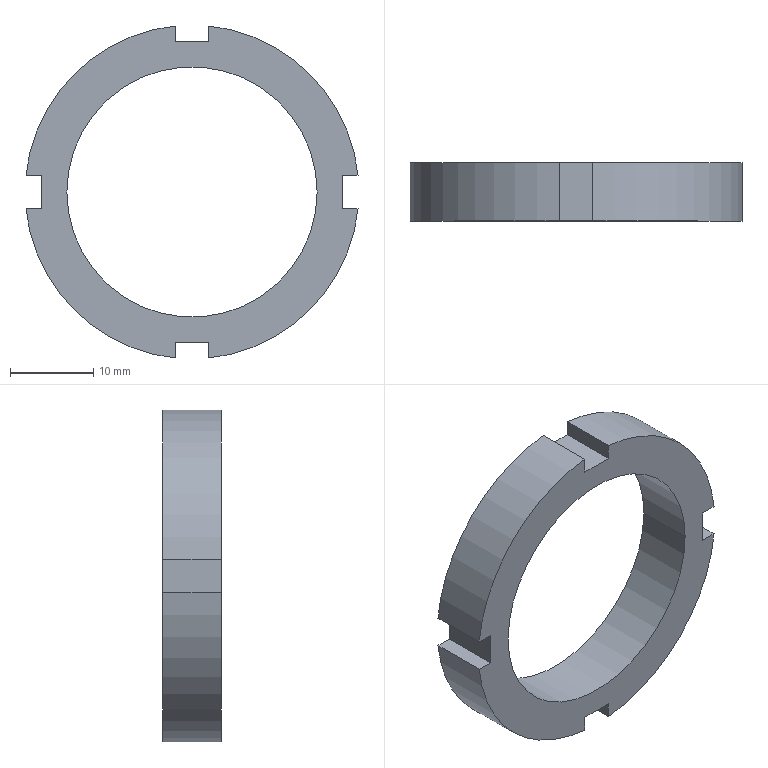Component | SolidWorks | -M30X1.5Nut-1 | 1 solid | 20 faces | box 39.8 x 7 x 39.8 mm | volume 3628 mm3 | plane 14 | cylinder 6 | commonest cylinder face diameters 40 x4 30 x2
build123d program:
from build123d import *

# Parameters (mm, degrees)
BOSS_EXTRUDE1_DEPTH        = 3.5
M30X2_0_TAPPED_HOLE1_D     = 30
M30X2_0_TAPPED_HOLE1_DEPTH = 70
M30X2_0_TAPPED_HOLE1_TIP   = 9.013


with BuildPart() as part:
    # Sketch1 → Boss-Extrude1 (new, symmetric)
    with BuildSketch(Plane.XY):
        with BuildLine():
            Line((2, 18), (2, 19.9))
            ThreePointArc((2, 19.9), (14.142, 14.142), (19.9, 2))
            Line((19.9, 2), (18, 2))
            Line((18, 2), (18, -2))
            Line((18, -2), (19.9, -2))
            ThreePointArc((19.9, -2), (14.142, -14.142), (2, -19.9))
            Line((2, -19.9), (2, -18))
            Line((2, -18), (-2, -18))
            Line((-2, -18), (-2, -19.9))
            ThreePointArc((-2, -19.9), (-14.142, -14.142), (-19.9, -2))
            Line((-19.9, -2), (-18, -2))
            Line((-18, -2), (-18, 2))
            Line((-18, 2), (-19.9, 2))
            ThreePointArc((-19.9, 2), (-14.142, 14.142), (-2, 19.9))
            Line((-2, 19.9), (-2, 18))
            Line((-2, 18), (2, 18))
        make_face()
    extrude(amount=BOSS_EXTRUDE1_DEPTH, both=True)

    # M30x2.0 Tapped Hole1
    with Locations(Plane.XY.offset(3.5)):
        with Locations((0, 0)):
            Hole(M30X2_0_TAPPED_HOLE1_D / 2, depth=M30X2_0_TAPPED_HOLE1_DEPTH)
            with Locations((0, 0, -(M30X2_0_TAPPED_HOLE1_DEPTH + M30X2_0_TAPPED_HOLE1_TIP / 2))):  # 118° drill point
                Cone(0, M30X2_0_TAPPED_HOLE1_D / 2, M30X2_0_TAPPED_HOLE1_TIP, mode=Mode.SUBTRACT)


solid = part.part

# Placed as in the assembly
solid = solid.moved(Location((205, 1325, -173), (90, 0, 0)))
STEP:
#1=COLOUR_RGB('',0.7922,0.8196,0.9333);
#2=FILL_AREA_STYLE_COLOUR('',#1);
#3=FILL_AREA_STYLE('',(#2));
#4=SURFACE_STYLE_FILL_AREA(#3);
#5=SURFACE_SIDE_STYLE('',(#4));
#6=SURFACE_STYLE_USAGE(.BOTH.,#5);
#7=PRESENTATION_STYLE_ASSIGNMENT((#6));
#8=CARTESIAN_POINT('',(7.48,52.303,-6.811));
#9=VERTEX_POINT('',#8);
#10=CARTESIAN_POINT('',(8.661,52.303,-6.811));
#11=VERTEX_POINT('',#10);
#12=CARTESIAN_POINT('',(8.071,52.303,-6.811));
#13=DIRECTION('',(0.,-1.,0.));
#14=DIRECTION('',(1.,0.,0.));
#15=AXIS2_PLACEMENT_3D('',#12,#13,#14);
#16=CIRCLE('',#15,0.5906);
#17=EDGE_CURVE('',#9,#11,#16,.T.);
#18=ORIENTED_EDGE('',*,*,#17,.F.);
#19=CARTESIAN_POINT('',(7.48,52.028,-6.811));
#20=VERTEX_POINT('',#19);
#21=CARTESIAN_POINT('',(7.48,52.028,-6.811));
#22=DIRECTION('',(0.,-1.,0.));
#23=VECTOR('',#22,39.37);
#24=LINE('',#21,#23);
#25=EDGE_CURVE('',#9,#20,#24,.T.);
#26=ORIENTED_EDGE('',*,*,#25,.T.);
#27=CARTESIAN_POINT('',(8.661,52.028,-6.811));
#28=VERTEX_POINT('',#27);
#29=CARTESIAN_POINT('',(8.071,52.028,-6.811));
#30=DIRECTION('',(0.,-1.,0.));
#31=DIRECTION('',(1.,0.,0.));
#32=AXIS2_PLACEMENT_3D('',#29,#30,#31);
#33=CIRCLE('',#32,0.5906);
#34=EDGE_CURVE('',#20,#28,#33,.T.);
#35=ORIENTED_EDGE('',*,*,#34,.T.);
#36=CARTESIAN_POINT('',(8.661,52.028,-6.811));
#37=DIRECTION('',(0.,-1.,0.));
#38=VECTOR('',#37,39.37);
#39=LINE('',#36,#38);
#40=EDGE_CURVE('',#11,#28,#39,.T.);
#41=ORIENTED_EDGE('',*,*,#40,.F.);
#42=EDGE_LOOP('',(#18,#26,#35,#41));
#43=FACE_OUTER_BOUND('',#42,.T.);
#44=CARTESIAN_POINT('',(8.071,52.028,-6.811));
#45=DIRECTION('',(0.,-1.,0.));
#46=DIRECTION('',(1.,0.,0.));
#47=AXIS2_PLACEMENT_3D('',#44,#45,#46);
#48=CYLINDRICAL_SURFACE('',#47,0.5906);
#49=ADVANCED_FACE('',(#43),#48,.F.);
#50=CARTESIAN_POINT('',(8.854,52.303,-6.732));
#51=VERTEX_POINT('',#50);
#52=CARTESIAN_POINT('',(8.15,52.303,-6.028));
#53=VERTEX_POINT('',#52);
#54=CARTESIAN_POINT('',(8.071,52.303,-6.811));
#55=DIRECTION('',(0.,-1.,0.));
#56=DIRECTION('',(1.,0.,0.));
#57=AXIS2_PLACEMENT_3D('',#54,#55,#56);
#58=CIRCLE('',#57,0.7874);
#59=EDGE_CURVE('',#51,#53,#58,.T.);
#60=ORIENTED_EDGE('',*,*,#59,.T.);
#61=CARTESIAN_POINT('',(8.15,52.028,-6.028));
#62=VERTEX_POINT('',#61);
#63=CARTESIAN_POINT('',(8.15,52.028,-6.028));
#64=DIRECTION('',(-0.,1.,-0.));
#65=VECTOR('',#64,39.37);
#66=LINE('',#63,#65);
#67=EDGE_CURVE('',#62,#53,#66,.T.);
#68=ORIENTED_EDGE('',*,*,#67,.F.);
#69=CARTESIAN_POINT('',(8.854,52.028,-6.732));
#70=VERTEX_POINT('',#69);
#71=CARTESIAN_POINT('',(8.071,52.028,-6.811));
#72=DIRECTION('',(0.,-1.,0.));
#73=DIRECTION('',(1.,0.,0.));
#74=AXIS2_PLACEMENT_3D('',#71,#72,#73);
#75=CIRCLE('',#74,0.7874);
#76=EDGE_CURVE('',#70,#62,#75,.T.);
#77=ORIENTED_EDGE('',*,*,#76,.F.);
#78=CARTESIAN_POINT('',(8.854,52.028,-6.732));
#79=DIRECTION('',(-0.,1.,-0.));
#80=VECTOR('',#79,39.37);
#81=LINE('',#78,#80);
#82=EDGE_CURVE('',#70,#51,#81,.T.);
#83=ORIENTED_EDGE('',*,*,#82,.T.);
#84=EDGE_LOOP('',(#60,#68,#77,#83));
#85=FACE_OUTER_BOUND('',#84,.T.);
#86=CARTESIAN_POINT('',(8.071,52.028,-6.811));
#87=DIRECTION('',(-0.,1.,-0.));
#88=DIRECTION('',(-1.,0.,0.));
#89=AXIS2_PLACEMENT_3D('',#86,#87,#88);
#90=CYLINDRICAL_SURFACE('',#89,0.7874);
#91=ADVANCED_FACE('',(#85),#90,.T.);
#92=CARTESIAN_POINT('',(8.15,52.303,-6.102));
#93=VERTEX_POINT('',#92);
#94=CARTESIAN_POINT('',(8.15,52.303,-6.102));
#95=DIRECTION('',(-0.,-0.,-1.));
#96=VECTOR('',#95,39.37);
#97=LINE('',#94,#96);
#98=EDGE_CURVE('',#53,#93,#97,.T.);
#99=ORIENTED_EDGE('',*,*,#98,.T.);
#100=CARTESIAN_POINT('',(8.15,52.028,-6.102));
#101=VERTEX_POINT('',#100);
#102=CARTESIAN_POINT('',(8.15,52.028,-6.102));
#103=DIRECTION('',(-0.,1.,-0.));
#104=VECTOR('',#103,39.37);
#105=LINE('',#102,#104);
#106=EDGE_CURVE('',#101,#93,#105,.T.);
#107=ORIENTED_EDGE('',*,*,#106,.F.);
#108=CARTESIAN_POINT('',(8.15,52.028,-6.102));
#109=DIRECTION('',(-0.,-0.,-1.));
#110=VECTOR('',#109,39.37);
#111=LINE('',#108,#110);
#112=EDGE_CURVE('',#62,#101,#111,.T.);
#113=ORIENTED_EDGE('',*,*,#112,.F.);
#114=ORIENTED_EDGE('',*,*,#67,.T.);
#115=EDGE_LOOP('',(#99,#107,#113,#114));
#116=FACE_OUTER_BOUND('',#115,.T.);
#117=CARTESIAN_POINT('',(8.15,52.028,-6.102));
#118=DIRECTION('',(1.,0.,-0.));
#119=DIRECTION('',(-0.,1.,-0.));
#120=AXIS2_PLACEMENT_3D('',#117,#118,#119);
#121=PLANE('',#120);
#122=ADVANCED_FACE('',(#116),#121,.F.);
#123=CARTESIAN_POINT('',(7.992,52.303,-6.102));
#124=VERTEX_POINT('',#123);
#125=CARTESIAN_POINT('',(7.992,52.303,-6.102));
#126=DIRECTION('',(-1.,-0.,0.));
#127=VECTOR('',#126,39.37);
#128=LINE('',#125,#127);
#129=EDGE_CURVE('',#93,#124,#128,.T.);
#130=ORIENTED_EDGE('',*,*,#129,.T.);
#131=CARTESIAN_POINT('',(7.992,52.028,-6.102));
#132=VERTEX_POINT('',#131);
#133=CARTESIAN_POINT('',(7.992,52.028,-6.102));
#134=DIRECTION('',(-0.,1.,-0.));
#135=VECTOR('',#134,39.37);
#136=LINE('',#133,#135);
#137=EDGE_CURVE('',#132,#124,#136,.T.);
#138=ORIENTED_EDGE('',*,*,#137,.F.);
#139=CARTESIAN_POINT('',(7.992,52.028,-6.102));
#140=DIRECTION('',(-1.,-0.,0.));
#141=VECTOR('',#140,39.37);
#142=LINE('',#139,#141);
#143=EDGE_CURVE('',#101,#132,#142,.T.);
#144=ORIENTED_EDGE('',*,*,#143,.F.);
#145=ORIENTED_EDGE('',*,*,#106,.T.);
#146=EDGE_LOOP('',(#130,#138,#144,#145));
#147=FACE_OUTER_BOUND('',#146,.T.);
#148=CARTESIAN_POINT('',(7.992,52.028,-6.102));
#149=DIRECTION('',(-0.,-0.,-1.));
#150=DIRECTION('',(-0.,1.,-0.));
#151=AXIS2_PLACEMENT_3D('',#148,#149,#150);
#152=PLANE('',#151);
#153=ADVANCED_FACE('',(#147),#152,.F.);
#154=CARTESIAN_POINT('',(7.992,52.303,-6.028));
#155=VERTEX_POINT('',#154);
#156=CARTESIAN_POINT('',(7.992,52.303,-6.102));
#157=DIRECTION('',(0.,0.,1.));
#158=VECTOR('',#157,39.37);
#159=LINE('',#156,#158);
#160=EDGE_CURVE('',#124,#155,#159,.T.);
#161=ORIENTED_EDGE('',*,*,#160,.T.);
#162=CARTESIAN_POINT('',(7.992,52.028,-6.028));
#163=VERTEX_POINT('',#162);
#164=CARTESIAN_POINT('',(7.992,52.028,-6.028));
#165=DIRECTION('',(-0.,1.,-0.));
#166=VECTOR('',#165,39.37);
#167=LINE('',#164,#166);
#168=EDGE_CURVE('',#163,#155,#167,.T.);
#169=ORIENTED_EDGE('',*,*,#168,.F.);
#170=CARTESIAN_POINT('',(7.992,52.028,-6.102));
#171=DIRECTION('',(0.,0.,1.));
#172=VECTOR('',#171,39.37);
#173=LINE('',#170,#172);
#174=EDGE_CURVE('',#132,#163,#173,.T.);
#175=ORIENTED_EDGE('',*,*,#174,.F.);
#176=ORIENTED_EDGE('',*,*,#137,.T.);
#177=EDGE_LOOP('',(#161,#169,#175,#176));
#178=FACE_OUTER_BOUND('',#177,.T.);
#179=CARTESIAN_POINT('',(7.992,52.028,-6.102));
#180=DIRECTION('',(-1.,-0.,0.));
#181=DIRECTION('',(0.,-1.,0.));
#182=AXIS2_PLACEMENT_3D('',#179,#180,#181);
#183=PLANE('',#182);
#184=ADVANCED_FACE('',(#178),#183,.F.);
#185=CARTESIAN_POINT('',(7.287,52.303,-6.732));
#186=VERTEX_POINT('',#185);
#187=CARTESIAN_POINT('',(8.071,52.303,-6.811));
#188=DIRECTION('',(0.,-1.,0.));
#189=DIRECTION('',(1.,0.,0.));
#190=AXIS2_PLACEMENT_3D('',#187,#188,#189);
#191=CIRCLE('',#190,0.7874);
#192=EDGE_CURVE('',#155,#186,#191,.T.);
#193=ORIENTED_EDGE('',*,*,#192,.T.);
#194=CARTESIAN_POINT('',(7.287,52.028,-6.732));
#195=VERTEX_POINT('',#194);
#196=CARTESIAN_POINT('',(7.287,52.028,-6.732));
#197=DIRECTION('',(-0.,1.,-0.));
#198=VECTOR('',#197,39.37);
#199=LINE('',#196,#198);
#200=EDGE_CURVE('',#195,#186,#199,.T.);
#201=ORIENTED_EDGE('',*,*,#200,.F.);
#202=CARTESIAN_POINT('',(8.071,52.028,-6.811));
#203=DIRECTION('',(0.,-1.,0.));
#204=DIRECTION('',(1.,0.,0.));
#205=AXIS2_PLACEMENT_3D('',#202,#203,#204);
#206=CIRCLE('',#205,0.7874);
#207=EDGE_CURVE('',#163,#195,#206,.T.);
#208=ORIENTED_EDGE('',*,*,#207,.F.);
#209=ORIENTED_EDGE('',*,*,#168,.T.);
#210=EDGE_LOOP('',(#193,#201,#208,#209));
#211=FACE_OUTER_BOUND('',#210,.T.);
#212=CARTESIAN_POINT('',(8.071,52.028,-6.811));
#213=DIRECTION('',(-0.,1.,-0.));
#214=DIRECTION('',(-1.,0.,0.));
#215=AXIS2_PLACEMENT_3D('',#212,#213,#214);
#216=CYLINDRICAL_SURFACE('',#215,0.7874);
#217=ADVANCED_FACE('',(#211),#216,.T.);
#218=CARTESIAN_POINT('',(7.362,52.303,-6.732));
#219=VERTEX_POINT('',#218);
#220=CARTESIAN_POINT('',(7.362,52.303,-6.732));
#221=DIRECTION('',(1.,0.,0.));
#222=VECTOR('',#221,39.37);
#223=LINE('',#220,#222);
#224=EDGE_CURVE('',#186,#219,#223,.T.);
#225=ORIENTED_EDGE('',*,*,#224,.T.);
#226=CARTESIAN_POINT('',(7.362,52.028,-6.732));
#227=VERTEX_POINT('',#226);
#228=CARTESIAN_POINT('',(7.362,52.028,-6.732));
#229=DIRECTION('',(-0.,1.,-0.));
#230=VECTOR('',#229,39.37);
#231=LINE('',#228,#230);
#232=EDGE_CURVE('',#227,#219,#231,.T.);
#233=ORIENTED_EDGE('',*,*,#232,.F.);
#234=CARTESIAN_POINT('',(7.362,52.028,-6.732));
#235=DIRECTION('',(1.,0.,0.));
#236=VECTOR('',#235,39.37);
#237=LINE('',#234,#236);
#238=EDGE_CURVE('',#195,#227,#237,.T.);
#239=ORIENTED_EDGE('',*,*,#238,.F.);
#240=ORIENTED_EDGE('',*,*,#200,.T.);
#241=EDGE_LOOP('',(#225,#233,#239,#240));
#242=FACE_OUTER_BOUND('',#241,.T.);
#243=CARTESIAN_POINT('',(7.362,52.028,-6.732));
#244=DIRECTION('',(-0.,0.,1.));
#245=DIRECTION('',(-1.,-0.,-0.));
#246=AXIS2_PLACEMENT_3D('',#243,#244,#245);
#247=PLANE('',#246);
#248=ADVANCED_FACE('',(#242),#247,.F.);
#249=CARTESIAN_POINT('',(7.362,52.303,-6.89));
#250=VERTEX_POINT('',#249);
#251=CARTESIAN_POINT('',(7.362,52.303,-6.89));
#252=DIRECTION('',(-0.,-0.,-1.));
#253=VECTOR('',#252,39.37);
#254=LINE('',#251,#253);
#255=EDGE_CURVE('',#219,#250,#254,.T.);
#256=ORIENTED_EDGE('',*,*,#255,.T.);
#257=CARTESIAN_POINT('',(7.362,52.028,-6.89));
#258=VERTEX_POINT('',#257);
#259=CARTESIAN_POINT('',(7.362,52.028,-6.89));
#260=DIRECTION('',(-0.,1.,-0.));
#261=VECTOR('',#260,39.37);
#262=LINE('',#259,#261);
#263=EDGE_CURVE('',#258,#250,#262,.T.);
#264=ORIENTED_EDGE('',*,*,#263,.F.);
#265=CARTESIAN_POINT('',(7.362,52.028,-6.89));
#266=DIRECTION('',(-0.,-0.,-1.));
#267=VECTOR('',#266,39.37);
#268=LINE('',#265,#267);
#269=EDGE_CURVE('',#227,#258,#268,.T.);
#270=ORIENTED_EDGE('',*,*,#269,.F.);
#271=ORIENTED_EDGE('',*,*,#232,.T.);
#272=EDGE_LOOP('',(#256,#264,#270,#271));
#273=FACE_OUTER_BOUND('',#272,.T.);
#274=CARTESIAN_POINT('',(7.362,52.028,-6.89));
#275=DIRECTION('',(1.,0.,-0.));
#276=DIRECTION('',(-0.,1.,-0.));
#277=AXIS2_PLACEMENT_3D('',#274,#275,#276);
#278=PLANE('',#277);
#279=ADVANCED_FACE('',(#273),#278,.F.);
#280=CARTESIAN_POINT('',(7.287,52.303,-6.89));
#281=VERTEX_POINT('',#280);
#282=CARTESIAN_POINT('',(7.362,52.303,-6.89));
#283=DIRECTION('',(-1.,-0.,-0.));
#284=VECTOR('',#283,39.37);
#285=LINE('',#282,#284);
#286=EDGE_CURVE('',#250,#281,#285,.T.);
#287=ORIENTED_EDGE('',*,*,#286,.T.);
#288=CARTESIAN_POINT('',(7.287,52.028,-6.89));
#289=VERTEX_POINT('',#288);
#290=CARTESIAN_POINT('',(7.287,52.028,-6.89));
#291=DIRECTION('',(-0.,1.,-0.));
#292=VECTOR('',#291,39.37);
#293=LINE('',#290,#292);
#294=EDGE_CURVE('',#289,#281,#293,.T.);
#295=ORIENTED_EDGE('',*,*,#294,.F.);
#296=CARTESIAN_POINT('',(7.362,52.028,-6.89));
#297=DIRECTION('',(-1.,-0.,-0.));
#298=VECTOR('',#297,39.37);
#299=LINE('',#296,#298);
#300=EDGE_CURVE('',#258,#289,#299,.T.);
#301=ORIENTED_EDGE('',*,*,#300,.F.);
#302=ORIENTED_EDGE('',*,*,#263,.T.);
#303=EDGE_LOOP('',(#287,#295,#301,#302));
#304=FACE_OUTER_BOUND('',#303,.T.);
#305=CARTESIAN_POINT('',(7.362,52.028,-6.89));
#306=DIRECTION('',(0.,-0.,-1.));
#307=DIRECTION('',(1.,0.,0.));
#308=AXIS2_PLACEMENT_3D('',#305,#306,#307);
#309=PLANE('',#308);
#310=ADVANCED_FACE('',(#304),#309,.F.);
#311=CARTESIAN_POINT('',(7.992,52.303,-7.594));
#312=VERTEX_POINT('',#311);
#313=CARTESIAN_POINT('',(8.071,52.303,-6.811));
#314=DIRECTION('',(0.,-1.,0.));
#315=DIRECTION('',(1.,0.,0.));
#316=AXIS2_PLACEMENT_3D('',#313,#314,#315);
#317=CIRCLE('',#316,0.7874);
#318=EDGE_CURVE('',#281,#312,#317,.T.);
#319=ORIENTED_EDGE('',*,*,#318,.T.);
#320=CARTESIAN_POINT('',(7.992,52.028,-7.594));
#321=VERTEX_POINT('',#320);
#322=CARTESIAN_POINT('',(7.992,52.028,-7.594));
#323=DIRECTION('',(-0.,1.,-0.));
#324=VECTOR('',#323,39.37);
#325=LINE('',#322,#324);
#326=EDGE_CURVE('',#321,#312,#325,.T.);
#327=ORIENTED_EDGE('',*,*,#326,.F.);
#328=CARTESIAN_POINT('',(8.071,52.028,-6.811));
#329=DIRECTION('',(0.,-1.,0.));
#330=DIRECTION('',(1.,0.,0.));
#331=AXIS2_PLACEMENT_3D('',#328,#329,#330);
#332=CIRCLE('',#331,0.7874);
#333=EDGE_CURVE('',#289,#321,#332,.T.);
#334=ORIENTED_EDGE('',*,*,#333,.F.);
#335=ORIENTED_EDGE('',*,*,#294,.T.);
#336=EDGE_LOOP('',(#319,#327,#334,#335));
#337=FACE_OUTER_BOUND('',#336,.T.);
#338=CARTESIAN_POINT('',(8.071,52.028,-6.811));
#339=DIRECTION('',(-0.,1.,-0.));
#340=DIRECTION('',(-1.,0.,0.));
#341=AXIS2_PLACEMENT_3D('',#338,#339,#340);
#342=CYLINDRICAL_SURFACE('',#341,0.7874);
#343=ADVANCED_FACE('',(#337),#342,.T.);
#344=CARTESIAN_POINT('',(7.992,52.303,-7.52));
#345=VERTEX_POINT('',#344);
#346=CARTESIAN_POINT('',(7.992,52.303,-7.52));
#347=DIRECTION('',(0.,0.,1.));
#348=VECTOR('',#347,39.37);
#349=LINE('',#346,#348);
#350=EDGE_CURVE('',#312,#345,#349,.T.);
#351=ORIENTED_EDGE('',*,*,#350,.T.);
#352=CARTESIAN_POINT('',(7.992,52.028,-7.52));
#353=VERTEX_POINT('',#352);
#354=CARTESIAN_POINT('',(7.992,52.028,-7.52));
#355=DIRECTION('',(-0.,1.,-0.));
#356=VECTOR('',#355,39.37);
#357=LINE('',#354,#356);
#358=EDGE_CURVE('',#353,#345,#357,.T.);
#359=ORIENTED_EDGE('',*,*,#358,.F.);
#360=CARTESIAN_POINT('',(7.992,52.028,-7.52));
#361=DIRECTION('',(0.,0.,1.));
#362=VECTOR('',#361,39.37);
#363=LINE('',#360,#362);
#364=EDGE_CURVE('',#321,#353,#363,.T.);
#365=ORIENTED_EDGE('',*,*,#364,.F.);
#366=ORIENTED_EDGE('',*,*,#326,.T.);
#367=EDGE_LOOP('',(#351,#359,#365,#366));
#368=FACE_OUTER_BOUND('',#367,.T.);
#369=CARTESIAN_POINT('',(7.992,52.028,-7.52));
#370=DIRECTION('',(-1.,-0.,0.));
#371=DIRECTION('',(0.,-1.,0.));
#372=AXIS2_PLACEMENT_3D('',#369,#370,#371);
#373=PLANE('',#372);
#374=ADVANCED_FACE('',(#368),#373,.F.);
#375=CARTESIAN_POINT('',(8.15,52.303,-7.52));
#376=VERTEX_POINT('',#375);
#377=CARTESIAN_POINT('',(8.15,52.303,-7.52));
#378=DIRECTION('',(1.,0.,-0.));
#379=VECTOR('',#378,39.37);
#380=LINE('',#377,#379);
#381=EDGE_CURVE('',#345,#376,#380,.T.);
#382=ORIENTED_EDGE('',*,*,#381,.T.);
#383=CARTESIAN_POINT('',(8.15,52.028,-7.52));
#384=VERTEX_POINT('',#383);
#385=CARTESIAN_POINT('',(8.15,52.028,-7.52));
#386=DIRECTION('',(-0.,1.,-0.));
#387=VECTOR('',#386,39.37);
#388=LINE('',#385,#387);
#389=EDGE_CURVE('',#384,#376,#388,.T.);
#390=ORIENTED_EDGE('',*,*,#389,.F.);
#391=CARTESIAN_POINT('',(8.15,52.028,-7.52));
#392=DIRECTION('',(1.,0.,-0.));
#393=VECTOR('',#392,39.37);
#394=LINE('',#391,#393);
#395=EDGE_CURVE('',#353,#384,#394,.T.);
#396=ORIENTED_EDGE('',*,*,#395,.F.);
#397=ORIENTED_EDGE('',*,*,#358,.T.);
#398=EDGE_LOOP('',(#382,#390,#396,#397));
#399=FACE_OUTER_BOUND('',#398,.T.);
#400=CARTESIAN_POINT('',(8.15,52.028,-7.52));
#401=DIRECTION('',(0.,0.,1.));
#402=DIRECTION('',(0.,-1.,0.));
#403=AXIS2_PLACEMENT_3D('',#400,#401,#402);
#404=PLANE('',#403);
#405=ADVANCED_FACE('',(#399),#404,.F.);
#406=CARTESIAN_POINT('',(8.15,52.303,-7.594));
#407=VERTEX_POINT('',#406);
#408=CARTESIAN_POINT('',(8.15,52.303,-7.52));
#409=DIRECTION('',(-0.,-0.,-1.));
#410=VECTOR('',#409,39.37);
#411=LINE('',#408,#410);
#412=EDGE_CURVE('',#376,#407,#411,.T.);
#413=ORIENTED_EDGE('',*,*,#412,.T.);
#414=CARTESIAN_POINT('',(8.15,52.028,-7.594));
#415=VERTEX_POINT('',#414);
#416=CARTESIAN_POINT('',(8.15,52.028,-7.594));
#417=DIRECTION('',(-0.,1.,-0.));
#418=VECTOR('',#417,39.37);
#419=LINE('',#416,#418);
#420=EDGE_CURVE('',#415,#407,#419,.T.);
#421=ORIENTED_EDGE('',*,*,#420,.F.);
#422=CARTESIAN_POINT('',(8.15,52.028,-7.52));
#423=DIRECTION('',(-0.,-0.,-1.));
#424=VECTOR('',#423,39.37);
#425=LINE('',#422,#424);
#426=EDGE_CURVE('',#384,#415,#425,.T.);
#427=ORIENTED_EDGE('',*,*,#426,.F.);
#428=ORIENTED_EDGE('',*,*,#389,.T.);
#429=EDGE_LOOP('',(#413,#421,#427,#428));
#430=FACE_OUTER_BOUND('',#429,.T.);
#431=CARTESIAN_POINT('',(8.15,52.028,-7.52));
#432=DIRECTION('',(1.,0.,-0.));
#433=DIRECTION('',(-0.,1.,-0.));
#434=AXIS2_PLACEMENT_3D('',#431,#432,#433);
#435=PLANE('',#434);
#436=ADVANCED_FACE('',(#430),#435,.F.);
#437=CARTESIAN_POINT('',(8.854,52.303,-6.89));
#438=VERTEX_POINT('',#437);
#439=CARTESIAN_POINT('',(8.071,52.303,-6.811));
#440=DIRECTION('',(0.,-1.,0.));
#441=DIRECTION('',(1.,0.,0.));
#442=AXIS2_PLACEMENT_3D('',#439,#440,#441);
#443=CIRCLE('',#442,0.7874);
#444=EDGE_CURVE('',#407,#438,#443,.T.);
#445=ORIENTED_EDGE('',*,*,#444,.T.);
#446=CARTESIAN_POINT('',(8.854,52.028,-6.89));
#447=VERTEX_POINT('',#446);
#448=CARTESIAN_POINT('',(8.854,52.028,-6.89));
#449=DIRECTION('',(-0.,1.,-0.));
#450=VECTOR('',#449,39.37);
#451=LINE('',#448,#450);
#452=EDGE_CURVE('',#447,#438,#451,.T.);
#453=ORIENTED_EDGE('',*,*,#452,.F.);
#454=CARTESIAN_POINT('',(8.071,52.028,-6.811));
#455=DIRECTION('',(0.,-1.,0.));
#456=DIRECTION('',(1.,0.,0.));
#457=AXIS2_PLACEMENT_3D('',#454,#455,#456);
#458=CIRCLE('',#457,0.7874);
#459=EDGE_CURVE('',#415,#447,#458,.T.);
#460=ORIENTED_EDGE('',*,*,#459,.F.);
#461=ORIENTED_EDGE('',*,*,#420,.T.);
#462=EDGE_LOOP('',(#445,#453,#460,#461));
#463=FACE_OUTER_BOUND('',#462,.T.);
#464=CARTESIAN_POINT('',(8.071,52.028,-6.811));
#465=DIRECTION('',(-0.,1.,-0.));
#466=DIRECTION('',(-1.,0.,0.));
#467=AXIS2_PLACEMENT_3D('',#464,#465,#466);
#468=CYLINDRICAL_SURFACE('',#467,0.7874);
#469=ADVANCED_FACE('',(#463),#468,.T.);
#470=CARTESIAN_POINT('',(8.78,52.303,-6.89));
#471=VERTEX_POINT('',#470);
#472=CARTESIAN_POINT('',(8.78,52.303,-6.89));
#473=DIRECTION('',(-1.,-0.,-0.));
#474=VECTOR('',#473,39.37);
#475=LINE('',#472,#474);
#476=EDGE_CURVE('',#438,#471,#475,.T.);
#477=ORIENTED_EDGE('',*,*,#476,.T.);
#478=CARTESIAN_POINT('',(8.78,52.028,-6.89));
#479=VERTEX_POINT('',#478);
#480=CARTESIAN_POINT('',(8.78,52.028,-6.89));
#481=DIRECTION('',(-0.,1.,-0.));
#482=VECTOR('',#481,39.37);
#483=LINE('',#480,#482);
#484=EDGE_CURVE('',#479,#471,#483,.T.);
#485=ORIENTED_EDGE('',*,*,#484,.F.);
#486=CARTESIAN_POINT('',(8.78,52.028,-6.89));
#487=DIRECTION('',(-1.,-0.,-0.));
#488=VECTOR('',#487,39.37);
#489=LINE('',#486,#488);
#490=EDGE_CURVE('',#447,#479,#489,.T.);
#491=ORIENTED_EDGE('',*,*,#490,.F.);
#492=ORIENTED_EDGE('',*,*,#452,.T.);
#493=EDGE_LOOP('',(#477,#485,#491,#492));
#494=FACE_OUTER_BOUND('',#493,.T.);
#495=CARTESIAN_POINT('',(8.78,52.028,-6.89));
#496=DIRECTION('',(0.,-0.,-1.));
#497=DIRECTION('',(1.,0.,0.));
#498=AXIS2_PLACEMENT_3D('',#495,#496,#497);
#499=PLANE('',#498);
#500=ADVANCED_FACE('',(#494),#499,.F.);
#501=CARTESIAN_POINT('',(8.78,52.303,-6.732));
#502=VERTEX_POINT('',#501);
#503=CARTESIAN_POINT('',(8.78,52.303,-6.732));
#504=DIRECTION('',(0.,0.,1.));
#505=VECTOR('',#504,39.37);
#506=LINE('',#503,#505);
#507=EDGE_CURVE('',#471,#502,#506,.T.);
#508=ORIENTED_EDGE('',*,*,#507,.T.);
#509=CARTESIAN_POINT('',(8.78,52.028,-6.732));
#510=VERTEX_POINT('',#509);
#511=CARTESIAN_POINT('',(8.78,52.028,-6.732));
#512=DIRECTION('',(-0.,1.,-0.));
#513=VECTOR('',#512,39.37);
#514=LINE('',#511,#513);
#515=EDGE_CURVE('',#510,#502,#514,.T.);
#516=ORIENTED_EDGE('',*,*,#515,.F.);
#517=CARTESIAN_POINT('',(8.78,52.028,-6.732));
#518=DIRECTION('',(0.,0.,1.));
#519=VECTOR('',#518,39.37);
#520=LINE('',#517,#519);
#521=EDGE_CURVE('',#479,#510,#520,.T.);
#522=ORIENTED_EDGE('',*,*,#521,.F.);
#523=ORIENTED_EDGE('',*,*,#484,.T.);
#524=EDGE_LOOP('',(#508,#516,#522,#523));
#525=FACE_OUTER_BOUND('',#524,.T.);
#526=CARTESIAN_POINT('',(8.78,52.028,-6.732));
#527=DIRECTION('',(-1.,-0.,0.));
#528=DIRECTION('',(0.,-1.,0.));
#529=AXIS2_PLACEMENT_3D('',#526,#527,#528);
#530=PLANE('',#529);
#531=ADVANCED_FACE('',(#525),#530,.F.);
#532=CARTESIAN_POINT('',(8.78,52.303,-6.732));
#533=DIRECTION('',(1.,0.,0.));
#534=VECTOR('',#533,39.37);
#535=LINE('',#532,#534);
#536=EDGE_CURVE('',#502,#51,#535,.T.);
#537=ORIENTED_EDGE('',*,*,#536,.T.);
#538=ORIENTED_EDGE('',*,*,#82,.F.);
#539=CARTESIAN_POINT('',(8.78,52.028,-6.732));
#540=DIRECTION('',(1.,0.,0.));
#541=VECTOR('',#540,39.37);
#542=LINE('',#539,#541);
#543=EDGE_CURVE('',#510,#70,#542,.T.);
#544=ORIENTED_EDGE('',*,*,#543,.F.);
#545=ORIENTED_EDGE('',*,*,#515,.T.);
#546=EDGE_LOOP('',(#537,#538,#544,#545));
#547=FACE_OUTER_BOUND('',#546,.T.);
#548=CARTESIAN_POINT('',(8.78,52.028,-6.732));
#549=DIRECTION('',(-0.,0.,1.));
#550=DIRECTION('',(-1.,-0.,-0.));
#551=AXIS2_PLACEMENT_3D('',#548,#549,#550);
#552=PLANE('',#551);
#553=ADVANCED_FACE('',(#547),#552,.F.);
#554=CARTESIAN_POINT('',(8.071,52.028,-6.811));
#555=DIRECTION('',(0.,-1.,0.));
#556=DIRECTION('',(1.,0.,0.));
#557=AXIS2_PLACEMENT_3D('',#554,#555,#556);
#558=CIRCLE('',#557,0.5906);
#559=EDGE_CURVE('',#28,#20,#558,.T.);
#560=ORIENTED_EDGE('',*,*,#559,.F.);
#561=ORIENTED_EDGE('',*,*,#34,.F.);
#562=EDGE_LOOP('',(#560,#561));
#563=FACE_BOUND('',#562,.T.);
#564=ORIENTED_EDGE('',*,*,#76,.T.);
#565=ORIENTED_EDGE('',*,*,#112,.T.);
#566=ORIENTED_EDGE('',*,*,#143,.T.);
#567=ORIENTED_EDGE('',*,*,#174,.T.);
#568=ORIENTED_EDGE('',*,*,#207,.T.);
#569=ORIENTED_EDGE('',*,*,#238,.T.);
#570=ORIENTED_EDGE('',*,*,#269,.T.);
#571=ORIENTED_EDGE('',*,*,#300,.T.);
#572=ORIENTED_EDGE('',*,*,#333,.T.);
#573=ORIENTED_EDGE('',*,*,#364,.T.);
#574=ORIENTED_EDGE('',*,*,#395,.T.);
#575=ORIENTED_EDGE('',*,*,#426,.T.);
#576=ORIENTED_EDGE('',*,*,#459,.T.);
#577=ORIENTED_EDGE('',*,*,#490,.T.);
#578=ORIENTED_EDGE('',*,*,#521,.T.);
#579=ORIENTED_EDGE('',*,*,#543,.T.);
#580=EDGE_LOOP('',(#564,#565,#566,#567,#568,#569,#570,#571,#572,#573,#574,#575,#576,#577,#578,#579));
#581=FACE_OUTER_BOUND('',#580,.T.);
#582=CARTESIAN_POINT('',(8.071,52.028,-6.811));
#583=DIRECTION('',(0.,-1.,0.));
#584=DIRECTION('',(1.,0.,-0.));
#585=AXIS2_PLACEMENT_3D('',#582,#583,#584);
#586=PLANE('',#585);
#587=ADVANCED_FACE('',(#563,#581),#586,.T.);
#588=CARTESIAN_POINT('',(8.071,52.303,-6.811));
#589=DIRECTION('',(0.,-1.,0.));
#590=DIRECTION('',(1.,0.,0.));
#591=AXIS2_PLACEMENT_3D('',#588,#589,#590);
#592=CIRCLE('',#591,0.5906);
#593=EDGE_CURVE('',#11,#9,#592,.T.);
#594=ORIENTED_EDGE('',*,*,#593,.T.);
#595=ORIENTED_EDGE('',*,*,#17,.T.);
#596=EDGE_LOOP('',(#594,#595));
#597=FACE_BOUND('',#596,.T.);
#598=ORIENTED_EDGE('',*,*,#59,.F.);
#599=ORIENTED_EDGE('',*,*,#536,.F.);
#600=ORIENTED_EDGE('',*,*,#507,.F.);
#601=ORIENTED_EDGE('',*,*,#476,.F.);
#602=ORIENTED_EDGE('',*,*,#444,.F.);
#603=ORIENTED_EDGE('',*,*,#412,.F.);
#604=ORIENTED_EDGE('',*,*,#381,.F.);
#605=ORIENTED_EDGE('',*,*,#350,.F.);
#606=ORIENTED_EDGE('',*,*,#318,.F.);
#607=ORIENTED_EDGE('',*,*,#286,.F.);
#608=ORIENTED_EDGE('',*,*,#255,.F.);
#609=ORIENTED_EDGE('',*,*,#224,.F.);
#610=ORIENTED_EDGE('',*,*,#192,.F.);
#611=ORIENTED_EDGE('',*,*,#160,.F.);
#612=ORIENTED_EDGE('',*,*,#129,.F.);
#613=ORIENTED_EDGE('',*,*,#98,.F.);
#614=EDGE_LOOP('',(#598,#599,#600,#601,#602,#603,#604,#605,#606,#607,#608,#609,#610,#611,#612,#613));
#615=FACE_OUTER_BOUND('',#614,.T.);
#616=CARTESIAN_POINT('',(8.071,52.303,-6.811));
#617=DIRECTION('',(0.,-1.,0.));
#618=DIRECTION('',(1.,0.,-0.));
#619=AXIS2_PLACEMENT_3D('',#616,#617,#618);
#620=PLANE('',#619);
#621=ADVANCED_FACE('',(#597,#615),#620,.F.);
#622=ORIENTED_EDGE('',*,*,#25,.F.);
#623=ORIENTED_EDGE('',*,*,#593,.F.);
#624=ORIENTED_EDGE('',*,*,#40,.T.);
#625=ORIENTED_EDGE('',*,*,#559,.T.);
#626=EDGE_LOOP('',(#622,#623,#624,#625));
#627=FACE_OUTER_BOUND('',#626,.T.);
#628=CARTESIAN_POINT('',(8.071,52.028,-6.811));
#629=DIRECTION('',(0.,-1.,0.));
#630=DIRECTION('',(1.,0.,0.));
#631=AXIS2_PLACEMENT_3D('',#628,#629,#630);
#632=CYLINDRICAL_SURFACE('',#631,0.5906);
#633=ADVANCED_FACE('',(#627),#632,.F.);
#634=CLOSED_SHELL('',(#49,#91,#122,#153,#184,#217,#248,#279,#310,#343,#374,#405,#436,#469,#500,#531,#553,#587,#621,#633));
#635=MANIFOLD_SOLID_BREP('',#634);
#636=STYLED_ITEM('',(#7),#635);
#637=PRESENTATION_LAYER_ASSIGNMENT('','',(#636));
#638=CARTESIAN_POINT('',(0.,0.,0.));
#639=DIRECTION('',(0.,0.,1.));
#640=DIRECTION('',(1.,0.,0.));
#641=AXIS2_PLACEMENT_3D('',#638,#639,#640);
#642=(LENGTH_UNIT()NAMED_UNIT(*)SI_UNIT($,.METRE.));
#643=LENGTH_MEASURE_WITH_UNIT(LENGTH_MEASURE(0.0254),#642);
#644=DIMENSIONAL_EXPONENTS(1.,0.,0.,0.,0.,0.,0.);
#645=(CONVERSION_BASED_UNIT('',#643)LENGTH_UNIT()NAMED_UNIT(#644));
#646=UNCERTAINTY_MEASURE_WITH_UNIT(LENGTH_MEASURE(0.00001),#645,'','');
#647=(NAMED_UNIT(*)PLANE_ANGLE_UNIT()SI_UNIT($,.RADIAN.));
#648=(NAMED_UNIT(*)SI_UNIT($,.STERADIAN.)SOLID_ANGLE_UNIT());
#649=(GEOMETRIC_REPRESENTATION_CONTEXT(3)GLOBAL_UNCERTAINTY_ASSIGNED_CONTEXT((#646))GLOBAL_UNIT_ASSIGNED_CONTEXT((#645,#647,#648))REPRESENTATION_CONTEXT('',''));
#650=ADVANCED_BREP_SHAPE_REPRESENTATION('',(#635,#641),#649);
#651=(LENGTH_UNIT()NAMED_UNIT(*)SI_UNIT($,.METRE.));
#652=LENGTH_MEASURE_WITH_UNIT(LENGTH_MEASURE(0.0254),#651);
#653=DIMENSIONAL_EXPONENTS(1.,0.,0.,0.,0.,0.,0.);
#654=(CONVERSION_BASED_UNIT('',#652)LENGTH_UNIT()NAMED_UNIT(#653));
#655=UNCERTAINTY_MEASURE_WITH_UNIT(LENGTH_MEASURE(0.00001),#654,'','');
#656=(NAMED_UNIT(*)PLANE_ANGLE_UNIT()SI_UNIT($,.RADIAN.));
#657=(NAMED_UNIT(*)SI_UNIT($,.STERADIAN.)SOLID_ANGLE_UNIT());
#658=(GEOMETRIC_REPRESENTATION_CONTEXT(3)GLOBAL_UNCERTAINTY_ASSIGNED_CONTEXT((#655))GLOBAL_UNIT_ASSIGNED_CONTEXT((#654,#656,#657))REPRESENTATION_CONTEXT('',''));
#659=MECHANICAL_DESIGN_GEOMETRIC_PRESENTATION_REPRESENTATION('',(#636),#658);